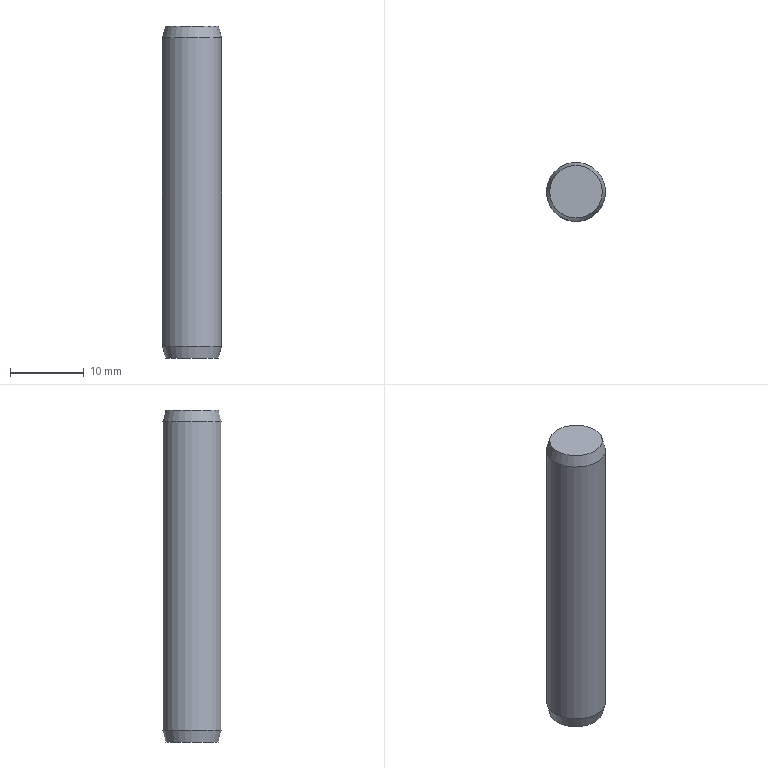Component | NX | GB-T119_1-2000_8X45 | 1 solid | 5 faces | box 8 x 8 x 45 mm | volume 2245 mm3 | plane 2 | cone 2 | cylinder 1 | commonest cylinder face diameters 8 x1
STEP:
#1=CARTESIAN_POINT('',(0.,0.,0.));
#2=DIRECTION('',(0.,0.,1.));
#3=DIRECTION('',(1.,0.,0.));
#4=AXIS2_PLACEMENT_3D('',#1,#2,#3);
#5=CARTESIAN_POINT('',(-13.571,144.033,35.));
#6=VERTEX_POINT('',#5);
#7=CARTESIAN_POINT('',(-10.,144.033,35.));
#8=DIRECTION('',(0.,0.,-1.));
#9=DIRECTION('',(-1.,0.,0.));
#10=AXIS2_PLACEMENT_3D('',#7,#8,#9);
#11=CIRCLE('',#10,3.571);
#12=CARTESIAN_POINT('',(-10.,144.033,35.));
#13=DIRECTION('',(0.,0.,-1.));
#14=DIRECTION('',(-1.,0.,0.));
#15=AXIS2_PLACEMENT_3D('',#12,#13,#14);
#16=PLANE('',#15);
#17=CARTESIAN_POINT('',(0.,0.));
#18=DIRECTION('',(1.,0.));
#19=AXIS2_PLACEMENT_2D('',#17,#18);
#20=CIRCLE('',#19,3.571);
#21=(GEOMETRIC_REPRESENTATION_CONTEXT(2)PARAMETRIC_REPRESENTATION_CONTEXT()REPRESENTATION_CONTEXT('',''));
#22=DEFINITIONAL_REPRESENTATION('',(#20),#21);
#23=PCURVE('',#16,#22);
#24=CARTESIAN_POINT('',(-10.,144.033,35.));
#25=DIRECTION('',(0.,0.,1.));
#26=DIRECTION('',(1.,0.,0.));
#27=AXIS2_PLACEMENT_3D('',#24,#25,#26);
#28=CONICAL_SURFACE('',#27,3.571,0.2618);
#29=CARTESIAN_POINT('',(9.425,0.));
#30=DIRECTION('',(-1.,0.));
#31=VECTOR('',#30,1.);
#32=LINE('',#29,#31);
#33=(GEOMETRIC_REPRESENTATION_CONTEXT(2)PARAMETRIC_REPRESENTATION_CONTEXT()REPRESENTATION_CONTEXT('',''));
#34=DEFINITIONAL_REPRESENTATION('',(#32),#33);
#35=PCURVE('',#28,#34);
#36=SURFACE_CURVE('',#11,(#23,#35),.PCURVE_S1.);
#37=EDGE_CURVE('',#6,#6,#36,.T.);
#38=ORIENTED_EDGE('',*,*,#37,.T.);
#39=EDGE_LOOP('',(#38));
#40=FACE_BOUND('',#39,.T.);
#41=ADVANCED_FACE('',(#40),#16,.T.);
#42=CARTESIAN_POINT('',(-14.,144.033,36.6));
#43=VERTEX_POINT('',#42);
#44=CARTESIAN_POINT('',(-10.,144.033,36.6));
#45=DIRECTION('',(0.,0.,-1.));
#46=DIRECTION('',(-1.,0.,0.));
#47=AXIS2_PLACEMENT_3D('',#44,#45,#46);
#48=CIRCLE('',#47,4.);
#49=CARTESIAN_POINT('',(9.425,1.6));
#50=DIRECTION('',(-1.,0.));
#51=VECTOR('',#50,1.);
#52=LINE('',#49,#51);
#53=(GEOMETRIC_REPRESENTATION_CONTEXT(2)PARAMETRIC_REPRESENTATION_CONTEXT()REPRESENTATION_CONTEXT('',''));
#54=DEFINITIONAL_REPRESENTATION('',(#52),#53);
#55=PCURVE('',#28,#54);
#56=CARTESIAN_POINT('',(-10.,144.033,80.));
#57=DIRECTION('',(0.,0.,-1.));
#58=DIRECTION('',(-1.,0.,0.));
#59=AXIS2_PLACEMENT_3D('',#56,#57,#58);
#60=CYLINDRICAL_SURFACE('',#59,4.);
#61=CARTESIAN_POINT('',(0.,43.4));
#62=DIRECTION('',(1.,0.));
#63=VECTOR('',#62,1.);
#64=LINE('',#61,#63);
#65=(GEOMETRIC_REPRESENTATION_CONTEXT(2)PARAMETRIC_REPRESENTATION_CONTEXT()REPRESENTATION_CONTEXT('',''));
#66=DEFINITIONAL_REPRESENTATION('',(#64),#65);
#67=PCURVE('',#60,#66);
#68=SURFACE_CURVE('',#48,(#55,#67),.PCURVE_S1.);
#69=EDGE_CURVE('',#43,#43,#68,.T.);
#70=ORIENTED_EDGE('',*,*,#69,.T.);
#71=CARTESIAN_POINT('',(-13.571,144.033,35.));
#72=CARTESIAN_POINT('',(-14.,144.033,36.6));
#73=B_SPLINE_CURVE_WITH_KNOTS('',1,(#71,#72),.UNSPECIFIED.,.F.,.F.,(2,2),(0.,1.656),.PIECEWISE_BEZIER_KNOTS.);
#74=CARTESIAN_POINT('',(3.142,0.));
#75=DIRECTION('',(0.,1.));
#76=VECTOR('',#75,1.);
#77=LINE('',#74,#76);
#78=(GEOMETRIC_REPRESENTATION_CONTEXT(2)PARAMETRIC_REPRESENTATION_CONTEXT()REPRESENTATION_CONTEXT('',''));
#79=DEFINITIONAL_REPRESENTATION('',(#77),#78);
#80=PCURVE('',#28,#79);
#81=CARTESIAN_POINT('',(9.425,0.));
#82=DIRECTION('',(0.,1.));
#83=VECTOR('',#82,1.);
#84=LINE('',#81,#83);
#85=(GEOMETRIC_REPRESENTATION_CONTEXT(2)PARAMETRIC_REPRESENTATION_CONTEXT()REPRESENTATION_CONTEXT('',''));
#86=DEFINITIONAL_REPRESENTATION('',(#84),#85);
#87=PCURVE('',#28,#86);
#88=SEAM_CURVE('',#73,(#80,#87),.PCURVE_S1.);
#89=EDGE_CURVE('',#6,#43,#88,.T.);
#90=ORIENTED_EDGE('',*,*,#89,.F.);
#91=ORIENTED_EDGE('',*,*,#37,.F.);
#92=ORIENTED_EDGE('',*,*,#89,.T.);
#93=EDGE_LOOP('',(#70,#90,#91,#92));
#94=FACE_BOUND('',#93,.T.);
#95=ADVANCED_FACE('',(#94),#28,.T.);
#96=CARTESIAN_POINT('',(-14.,144.033,78.4));
#97=VERTEX_POINT('',#96);
#98=CARTESIAN_POINT('',(-10.,144.033,78.4));
#99=DIRECTION('',(0.,0.,-1.));
#100=DIRECTION('',(-1.,0.,0.));
#101=AXIS2_PLACEMENT_3D('',#98,#99,#100);
#102=CIRCLE('',#101,4.);
#103=CARTESIAN_POINT('',(0.,1.6));
#104=DIRECTION('',(1.,0.));
#105=VECTOR('',#104,1.);
#106=LINE('',#103,#105);
#107=(GEOMETRIC_REPRESENTATION_CONTEXT(2)PARAMETRIC_REPRESENTATION_CONTEXT()REPRESENTATION_CONTEXT('',''));
#108=DEFINITIONAL_REPRESENTATION('',(#106),#107);
#109=PCURVE('',#60,#108);
#110=CARTESIAN_POINT('',(-10.,144.033,78.4));
#111=DIRECTION('',(0.,0.,-1.));
#112=DIRECTION('',(-1.,0.,0.));
#113=AXIS2_PLACEMENT_3D('',#110,#111,#112);
#114=CONICAL_SURFACE('',#113,4.,0.2618);
#115=CARTESIAN_POINT('',(0.,0.));
#116=DIRECTION('',(1.,0.));
#117=VECTOR('',#116,1.);
#118=LINE('',#115,#117);
#119=(GEOMETRIC_REPRESENTATION_CONTEXT(2)PARAMETRIC_REPRESENTATION_CONTEXT()REPRESENTATION_CONTEXT('',''));
#120=DEFINITIONAL_REPRESENTATION('',(#118),#119);
#121=PCURVE('',#114,#120);
#122=SURFACE_CURVE('',#102,(#109,#121),.PCURVE_S1.);
#123=EDGE_CURVE('',#97,#97,#122,.T.);
#124=ORIENTED_EDGE('',*,*,#123,.T.);
#125=CARTESIAN_POINT('',(-14.,144.033,78.4));
#126=CARTESIAN_POINT('',(-14.,144.033,36.6));
#127=B_SPLINE_CURVE_WITH_KNOTS('',1,(#125,#126),.UNSPECIFIED.,.F.,.F.,(2,2),(1.6,43.4),.PIECEWISE_BEZIER_KNOTS.);
#128=CARTESIAN_POINT('',(6.283,0.));
#129=DIRECTION('',(0.,1.));
#130=VECTOR('',#129,1.);
#131=LINE('',#128,#130);
#132=(GEOMETRIC_REPRESENTATION_CONTEXT(2)PARAMETRIC_REPRESENTATION_CONTEXT()REPRESENTATION_CONTEXT('',''));
#133=DEFINITIONAL_REPRESENTATION('',(#131),#132);
#134=PCURVE('',#60,#133);
#135=CARTESIAN_POINT('',(0.,0.));
#136=DIRECTION('',(0.,1.));
#137=VECTOR('',#136,1.);
#138=LINE('',#135,#137);
#139=(GEOMETRIC_REPRESENTATION_CONTEXT(2)PARAMETRIC_REPRESENTATION_CONTEXT()REPRESENTATION_CONTEXT('',''));
#140=DEFINITIONAL_REPRESENTATION('',(#138),#139);
#141=PCURVE('',#60,#140);
#142=SEAM_CURVE('',#127,(#134,#141),.PCURVE_S1.);
#143=EDGE_CURVE('',#97,#43,#142,.T.);
#144=ORIENTED_EDGE('',*,*,#143,.T.);
#145=ORIENTED_EDGE('',*,*,#69,.F.);
#146=ORIENTED_EDGE('',*,*,#143,.F.);
#147=EDGE_LOOP('',(#124,#144,#145,#146));
#148=FACE_BOUND('',#147,.T.);
#149=ADVANCED_FACE('',(#148),#60,.T.);
#150=CARTESIAN_POINT('',(-13.571,144.033,80.));
#151=VERTEX_POINT('',#150);
#152=CARTESIAN_POINT('',(-10.,144.033,80.));
#153=DIRECTION('',(0.,0.,-1.));
#154=DIRECTION('',(-1.,0.,0.));
#155=AXIS2_PLACEMENT_3D('',#152,#153,#154);
#156=CIRCLE('',#155,3.571);
#157=CARTESIAN_POINT('',(0.,-1.6));
#158=DIRECTION('',(1.,0.));
#159=VECTOR('',#158,1.);
#160=LINE('',#157,#159);
#161=(GEOMETRIC_REPRESENTATION_CONTEXT(2)PARAMETRIC_REPRESENTATION_CONTEXT()REPRESENTATION_CONTEXT('',''));
#162=DEFINITIONAL_REPRESENTATION('',(#160),#161);
#163=PCURVE('',#114,#162);
#164=CARTESIAN_POINT('',(-6.429,144.033,80.));
#165=DIRECTION('',(0.,0.,1.));
#166=DIRECTION('',(1.,0.,0.));
#167=AXIS2_PLACEMENT_3D('',#164,#165,#166);
#168=PLANE('',#167);
#169=CARTESIAN_POINT('',(-7.143,0.));
#170=CARTESIAN_POINT('',(-7.143,6.186));
#171=CARTESIAN_POINT('',(-1.786,3.093));
#172=CARTESIAN_POINT('',(3.571,0.));
#173=CARTESIAN_POINT('',(-1.786,-3.093));
#174=CARTESIAN_POINT('',(-7.143,-6.186));
#175=CARTESIAN_POINT('',(-7.143,0.));
#176=(BOUNDED_CURVE()B_SPLINE_CURVE(2,(#169,#170,#171,#172,#173,#174,#175),.UNSPECIFIED.,.T.,.F.)B_SPLINE_CURVE_WITH_KNOTS((1,2,2,2,2,1),(-2.094,0.,2.094,4.189,6.283,8.378),.UNSPECIFIED.)CURVE()GEOMETRIC_REPRESENTATION_ITEM()RATIONAL_B_SPLINE_CURVE((1.,0.5,1.,0.5,1.,0.5,1.))REPRESENTATION_ITEM(''));
#177=(GEOMETRIC_REPRESENTATION_CONTEXT(2)PARAMETRIC_REPRESENTATION_CONTEXT()REPRESENTATION_CONTEXT('',''));
#178=DEFINITIONAL_REPRESENTATION('',(#176),#177);
#179=PCURVE('',#168,#178);
#180=SURFACE_CURVE('',#156,(#163,#179),.PCURVE_S1.);
#181=EDGE_CURVE('',#151,#151,#180,.T.);
#182=ORIENTED_EDGE('',*,*,#181,.T.);
#183=CARTESIAN_POINT('',(-13.571,144.033,80.));
#184=CARTESIAN_POINT('',(-14.,144.033,78.4));
#185=B_SPLINE_CURVE_WITH_KNOTS('',1,(#183,#184),.UNSPECIFIED.,.F.,.F.,(2,2),(-1.656,0.),.PIECEWISE_BEZIER_KNOTS.);
#186=CARTESIAN_POINT('',(6.283,0.));
#187=DIRECTION('',(0.,1.));
#188=VECTOR('',#187,1.);
#189=LINE('',#186,#188);
#190=(GEOMETRIC_REPRESENTATION_CONTEXT(2)PARAMETRIC_REPRESENTATION_CONTEXT()REPRESENTATION_CONTEXT('',''));
#191=DEFINITIONAL_REPRESENTATION('',(#189),#190);
#192=PCURVE('',#114,#191);
#193=CARTESIAN_POINT('',(0.,0.));
#194=DIRECTION('',(0.,1.));
#195=VECTOR('',#194,1.);
#196=LINE('',#193,#195);
#197=(GEOMETRIC_REPRESENTATION_CONTEXT(2)PARAMETRIC_REPRESENTATION_CONTEXT()REPRESENTATION_CONTEXT('',''));
#198=DEFINITIONAL_REPRESENTATION('',(#196),#197);
#199=PCURVE('',#114,#198);
#200=SEAM_CURVE('',#185,(#192,#199),.PCURVE_S1.);
#201=EDGE_CURVE('',#151,#97,#200,.T.);
#202=ORIENTED_EDGE('',*,*,#201,.T.);
#203=ORIENTED_EDGE('',*,*,#123,.F.);
#204=ORIENTED_EDGE('',*,*,#201,.F.);
#205=EDGE_LOOP('',(#182,#202,#203,#204));
#206=FACE_BOUND('',#205,.T.);
#207=ADVANCED_FACE('',(#206),#114,.T.);
#208=ORIENTED_EDGE('',*,*,#181,.F.);
#209=EDGE_LOOP('',(#208));
#210=FACE_BOUND('',#209,.T.);
#211=ADVANCED_FACE('',(#210),#168,.T.);
#212=CLOSED_SHELL('',(#41,#95,#149,#207,#211));
#213=MANIFOLD_SOLID_BREP('',#212);
#214=(LENGTH_UNIT()NAMED_UNIT(*)SI_UNIT(.MILLI.,.METRE.));
#215=UNCERTAINTY_MEASURE_WITH_UNIT(LENGTH_MEASURE(0.00001),#214,'','');
#216=(NAMED_UNIT(*)PLANE_ANGLE_UNIT()SI_UNIT($,.RADIAN.));
#217=(NAMED_UNIT(*)SI_UNIT($,.STERADIAN.)SOLID_ANGLE_UNIT());
#218=(GEOMETRIC_REPRESENTATION_CONTEXT(3)GLOBAL_UNCERTAINTY_ASSIGNED_CONTEXT((#215))GLOBAL_UNIT_ASSIGNED_CONTEXT((#214,#216,#217))REPRESENTATION_CONTEXT('',''));
#219=ADVANCED_BREP_SHAPE_REPRESENTATION('',(#4,#213),#218);